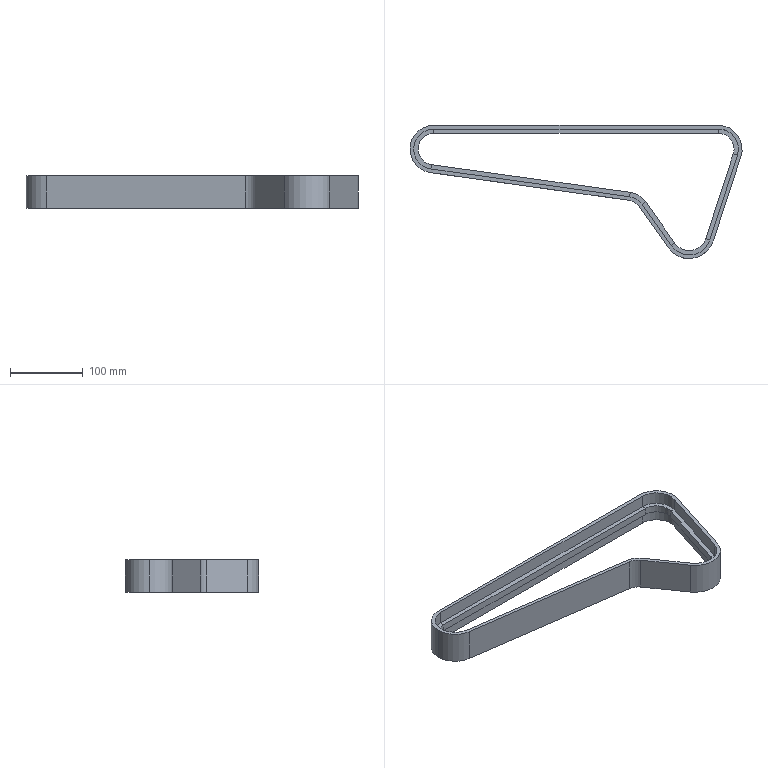Component | SolidWorks | 170423A4-Belt-1 | 1 solid | 54 faces | box 455 x 182.5 x 45 mm | volume 309436 mm3 | plane 34 | cylinder 20 | commonest cylinder face diameters 55 x6 43 x3 65 x3 50 x2 60 x2 40 x1 70 x1 62 x1
build123d program:
from build123d import *

# Parameters (mm, degrees)
BOSS_EXTRUDE1_DEPTH = 45
SKETCH2_W           = 10
SKETCH2_H           = 6


with BuildPart() as part:
    # Sketch1 → Boss-Extrude1 (new body)
    with BuildSketch(Plane.XY):
        with BuildLine():
            Line((0, 32.5), (390, 32.5))
            ThreePointArc((390, 32.5), (416.293, 19.102), (420.909, -10.044))
            Line((420.909, -10.044), (383.287, -125.817))
            ThreePointArc((383.287, -125.817), (355.245, -149.605), (321.413, -135.194))
            Line((321.413, -135.194), (281.335, -78.46))
            ThreePointArc((281.335, -78.46), (275.407, -72.921), (267.765, -70.192))
            Line((267.765, -70.192), (-4.493, -32.188))
            ThreePointArc((-4.493, -32.188), (-32.422, 2.252), (0, 32.5))
        make_face()
        with BuildLine():
            Line((0, 27.5), (390, 27.5))
            ThreePointArc((390, 27.5), (412.248, 16.164), (416.154, -8.499))
            Line((416.154, -8.499), (378.531, -124.272))
            ThreePointArc((378.531, -124.272), (354.495, -144.661), (325.497, -132.309))
            Line((325.497, -132.309), (285.419, -75.576))
            ThreePointArc((285.419, -75.576), (278.008, -68.651), (268.456, -65.24))
            Line((268.456, -65.24), (-3.802, -27.236))
            ThreePointArc((-3.802, -27.236), (-27.434, 1.905), (0, 27.5))
        make_face(mode=Mode.SUBTRACT)
    extrude(amount=BOSS_EXTRUDE1_DEPTH)

    # Sweep1: sweep along a path in Sketch3
    with BuildLine(Plane.XY.offset(22.5)) as sweep1_path:
        Line((-3.802, -27.236), (268.456, -65.24))
        ThreePointArc((268.456, -65.24), (278.008, -68.651), (285.419, -75.576))
        Line((285.419, -75.576), (325.497, -132.309))
        ThreePointArc((325.497, -132.309), (354.495, -144.661), (378.531, -124.272))
        Line((378.531, -124.272), (416.154, -8.499))
        ThreePointArc((416.154, -8.499), (412.248, 16.164), (390, 27.5))
        Line((390, 27.5), (0, 27.5))
        ThreePointArc((0, 27.5), (-27.434, 1.905), (-3.802, -27.236))
    # Sketch2 → Sweep1 (sweep)
    with BuildSketch(Plane(origin=(0, 0, 0), x_dir=(0, 0, -1), z_dir=(1, 0, 0))):
        with Locations((-22.5, 24.5)):
            Rectangle(SKETCH2_W, SKETCH2_H)
    sweep(path=sweep1_path.line)


solid = part.part

# Placed as in the assembly
solid = solid.moved(Location((-250.246, -5.788, 421.5), (0, 0, 0)))